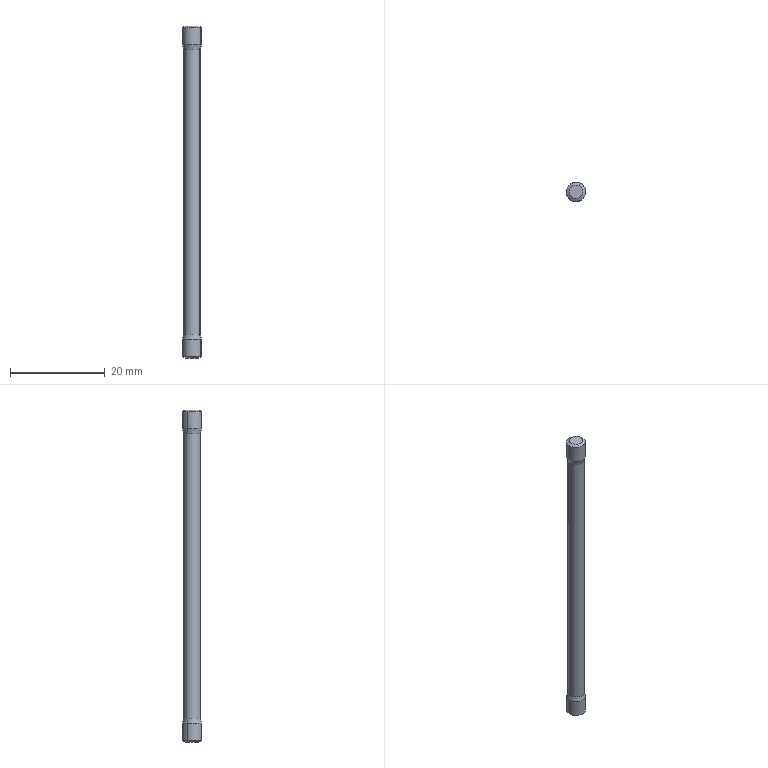Component | SolidWorks | GB_T901-1988EqualLengthDoubleEndStudGradeBM4x70-1 | 1 solid | 16 faces | box 4 x 4 x 70 mm | volume 685 mm3 | cone 8 | cylinder 6 | plane 2 | commonest cylinder face diameters 4 x4 3.464 x2
build123d program:
from build123d import *


with BuildPart() as part:
    # Sketch1 → Base-Revolve (revolve)
    with BuildSketch(Plane.XY, mode=Mode.PRIVATE) as base_revolve_sk:
        Polygon((-35, 2), (-31, 2), (-30.02, 1.732), (0, 1.732), (0, 0), (-35, 0), align=None)
    revolve(base_revolve_sk.sketch.rotate(Axis((-35, 0, 0), (1, 0, 0)), 180), axis=Axis((-35, 0, 0), (1, 0, 0)))

    # Sketch2 → Thread Cut (revolve, cut)
    with BuildSketch(Plane.XY, mode=Mode.PRIVATE) as thread_cut_sk:
        Polygon((-35.35, 2), (-34.65, 2), (-35, 1.394), align=None)
    revolve(thread_cut_sk.sketch.rotate(Axis((-26.952, 0, 0), (1, 0, 0)), 180), axis=Axis((-26.952, 0, 0), (1, 0, 0)), mode=Mode.SUBTRACT)

    # Mirror All1: part across plane


with BuildPart() as part_1:
    add(part.part)
    add(part.part.mirror(Plane(origin=(0, 1.732, 0), x_dir=(0, 0, 1), z_dir=(-1, 0, 0))))


solid = part_1.part

# Placed as in the assembly
solid = solid.moved(Location((-5.875, 10.354, 22.484), (0, 90, 0)))
STEP:
#1=COLOUR_RGB('',0.7922,0.8196,0.9333);
#2=FILL_AREA_STYLE_COLOUR('',#1);
#3=FILL_AREA_STYLE('',(#2));
#4=SURFACE_STYLE_FILL_AREA(#3);
#5=SURFACE_SIDE_STYLE('',(#4));
#6=SURFACE_STYLE_USAGE(.BOTH.,#5);
#7=PRESENTATION_STYLE_ASSIGNMENT((#6));
#8=CARTESIAN_POINT('',(-0.2571,0.3592,2.263));
#9=VERTEX_POINT('',#8);
#10=CARTESIAN_POINT('',(-0.2055,0.456,2.263));
#11=VERTEX_POINT('',#10);
#12=CARTESIAN_POINT('',(-0.2313,0.4076,2.263));
#13=DIRECTION('',(0.,0.,-1.));
#14=DIRECTION('',(0.4702,0.8826,0.));
#15=AXIS2_PLACEMENT_3D('',#12,#13,#14);
#16=CIRCLE('',#15,0.05487);
#17=EDGE_CURVE('',#9,#11,#16,.T.);
#18=ORIENTED_EDGE('',*,*,#17,.T.);
#19=CARTESIAN_POINT('',(-0.1943,0.4771,2.249));
#20=VERTEX_POINT('',#19);
#21=CARTESIAN_POINT('',(-0.2055,0.456,2.263));
#22=DIRECTION('',(0.4072,0.7643,-0.5));
#23=VECTOR('',#22,39.37);
#24=LINE('',#21,#23);
#25=EDGE_CURVE('',#11,#20,#24,.T.);
#26=ORIENTED_EDGE('',*,*,#25,.T.);
#27=CARTESIAN_POINT('',(-0.3008,0.4446,2.249));
#28=VERTEX_POINT('',#27);
#29=CARTESIAN_POINT('',(-0.2313,0.4076,2.249));
#30=DIRECTION('',(0.,0.,-1.));
#31=DIRECTION('',(0.4702,0.8826,0.));
#32=AXIS2_PLACEMENT_3D('',#29,#30,#31);
#33=CIRCLE('',#32,0.07874);
#34=EDGE_CURVE('',#28,#20,#33,.T.);
#35=ORIENTED_EDGE('',*,*,#34,.F.);
#36=CARTESIAN_POINT('',(-0.2683,0.3381,2.249));
#37=VERTEX_POINT('',#36);
#38=CARTESIAN_POINT('',(-0.2313,0.4076,2.249));
#39=DIRECTION('',(0.,0.,-1.));
#40=DIRECTION('',(0.4702,0.8826,0.));
#41=AXIS2_PLACEMENT_3D('',#38,#39,#40);
#42=CIRCLE('',#41,0.07874);
#43=EDGE_CURVE('',#37,#28,#42,.T.);
#44=ORIENTED_EDGE('',*,*,#43,.F.);
#45=CARTESIAN_POINT('',(-0.2571,0.3592,2.263));
#46=DIRECTION('',(-0.4072,-0.7643,-0.5));
#47=VECTOR('',#46,39.37);
#48=LINE('',#45,#47);
#49=EDGE_CURVE('',#9,#37,#48,.T.);
#50=ORIENTED_EDGE('',*,*,#49,.F.);
#51=EDGE_LOOP('',(#18,#26,#35,#44,#50));
#52=FACE_OUTER_BOUND('',#51,.T.);
#53=CARTESIAN_POINT('',(-0.2313,0.4076,2.263));
#54=DIRECTION('',(0.,0.,-1.));
#55=DIRECTION('',(-0.4702,-0.8826,0.));
#56=AXIS2_PLACEMENT_3D('',#53,#54,#55);
#57=CONICAL_SURFACE('',#56,0.05487,1.047);
#58=ADVANCED_FACE('',(#52),#57,.T.);
#59=CARTESIAN_POINT('',(-0.1711,0.3756,2.067));
#60=VERTEX_POINT('',#59);
#61=CARTESIAN_POINT('',(-0.2915,0.4397,2.067));
#62=VERTEX_POINT('',#61);
#63=CARTESIAN_POINT('',(-0.2313,0.4076,2.067));
#64=DIRECTION('',(0.,0.,-1.));
#65=DIRECTION('',(-0.8826,0.4702,0.));
#66=AXIS2_PLACEMENT_3D('',#63,#64,#65);
#67=CIRCLE('',#66,0.06819);
#68=EDGE_CURVE('',#60,#62,#67,.T.);
#69=ORIENTED_EDGE('',*,*,#68,.F.);
#70=CARTESIAN_POINT('',(-0.1618,0.3706,2.106));
#71=VERTEX_POINT('',#70);
#72=CARTESIAN_POINT('',(-0.1711,0.3756,2.067));
#73=DIRECTION('',(0.2328,-0.124,0.9646));
#74=VECTOR('',#73,39.37);
#75=LINE('',#72,#74);
#76=EDGE_CURVE('',#60,#71,#75,.T.);
#77=ORIENTED_EDGE('',*,*,#76,.T.);
#78=CARTESIAN_POINT('',(-0.3008,0.4446,2.106));
#79=VERTEX_POINT('',#78);
#80=CARTESIAN_POINT('',(-0.2313,0.4076,2.106));
#81=DIRECTION('',(0.,0.,-1.));
#82=DIRECTION('',(-0.8826,0.4702,0.));
#83=AXIS2_PLACEMENT_3D('',#80,#81,#82);
#84=CIRCLE('',#83,0.07874);
#85=EDGE_CURVE('',#71,#79,#84,.T.);
#86=ORIENTED_EDGE('',*,*,#85,.T.);
#87=CARTESIAN_POINT('',(-0.2915,0.4397,2.067));
#88=DIRECTION('',(-0.2328,0.124,0.9646));
#89=VECTOR('',#88,39.37);
#90=LINE('',#87,#89);
#91=EDGE_CURVE('',#62,#79,#90,.T.);
#92=ORIENTED_EDGE('',*,*,#91,.F.);
#93=EDGE_LOOP('',(#69,#77,#86,#92));
#94=FACE_OUTER_BOUND('',#93,.T.);
#95=CARTESIAN_POINT('',(-0.2313,0.4076,2.067));
#96=DIRECTION('',(-0.,-0.,1.));
#97=DIRECTION('',(-0.8826,0.4702,0.));
#98=AXIS2_PLACEMENT_3D('',#95,#96,#97);
#99=CONICAL_SURFACE('',#98,0.06819,0.2669);
#100=ADVANCED_FACE('',(#94),#99,.T.);
#101=ORIENTED_EDGE('',*,*,#85,.F.);
#102=CARTESIAN_POINT('',(-0.1618,0.3706,2.249));
#103=VERTEX_POINT('',#102);
#104=CARTESIAN_POINT('',(-0.1618,0.3706,2.263));
#105=DIRECTION('',(-0.,-0.,1.));
#106=VECTOR('',#105,39.37);
#107=LINE('',#104,#106);
#108=EDGE_CURVE('',#71,#103,#107,.T.);
#109=ORIENTED_EDGE('',*,*,#108,.T.);
#110=CARTESIAN_POINT('',(-0.2313,0.4076,2.249));
#111=DIRECTION('',(0.,0.,-1.));
#112=DIRECTION('',(0.4702,0.8826,0.));
#113=AXIS2_PLACEMENT_3D('',#110,#111,#112);
#114=CIRCLE('',#113,0.07874);
#115=EDGE_CURVE('',#103,#37,#114,.T.);
#116=ORIENTED_EDGE('',*,*,#115,.T.);
#117=ORIENTED_EDGE('',*,*,#43,.T.);
#118=CARTESIAN_POINT('',(-0.3008,0.4446,2.263));
#119=DIRECTION('',(-0.,-0.,1.));
#120=VECTOR('',#119,39.37);
#121=LINE('',#118,#120);
#122=EDGE_CURVE('',#79,#28,#121,.T.);
#123=ORIENTED_EDGE('',*,*,#122,.F.);
#124=EDGE_LOOP('',(#101,#109,#116,#117,#123));
#125=FACE_OUTER_BOUND('',#124,.T.);
#126=CARTESIAN_POINT('',(-0.2313,0.4076,2.263));
#127=DIRECTION('',(-0.,-0.,1.));
#128=DIRECTION('',(-0.8826,0.4702,0.));
#129=AXIS2_PLACEMENT_3D('',#126,#127,#128);
#130=CYLINDRICAL_SURFACE('',#129,0.07874);
#131=ADVANCED_FACE('',(#125),#130,.T.);
#132=CARTESIAN_POINT('',(-0.2055,0.456,-0.4928));
#133=VERTEX_POINT('',#132);
#134=CARTESIAN_POINT('',(-0.2571,0.3592,-0.4928));
#135=VERTEX_POINT('',#134);
#136=CARTESIAN_POINT('',(-0.2313,0.4076,-0.4928));
#137=DIRECTION('',(0.,0.,-1.));
#138=DIRECTION('',(0.4702,0.8826,0.));
#139=AXIS2_PLACEMENT_3D('',#136,#137,#138);
#140=CIRCLE('',#139,0.05487);
#141=EDGE_CURVE('',#133,#135,#140,.T.);
#142=ORIENTED_EDGE('',*,*,#141,.F.);
#143=CARTESIAN_POINT('',(-0.1943,0.4771,-0.479));
#144=VERTEX_POINT('',#143);
#145=CARTESIAN_POINT('',(-0.2055,0.456,-0.4928));
#146=DIRECTION('',(0.4072,0.7643,0.5));
#147=VECTOR('',#146,39.37);
#148=LINE('',#145,#147);
#149=EDGE_CURVE('',#133,#144,#148,.T.);
#150=ORIENTED_EDGE('',*,*,#149,.T.);
#151=CARTESIAN_POINT('',(-0.1618,0.3706,-0.479));
#152=VERTEX_POINT('',#151);
#153=CARTESIAN_POINT('',(-0.2313,0.4076,-0.479));
#154=DIRECTION('',(0.,0.,-1.));
#155=DIRECTION('',(0.4702,0.8826,0.));
#156=AXIS2_PLACEMENT_3D('',#153,#154,#155);
#157=CIRCLE('',#156,0.07874);
#158=EDGE_CURVE('',#144,#152,#157,.T.);
#159=ORIENTED_EDGE('',*,*,#158,.T.);
#160=CARTESIAN_POINT('',(-0.2683,0.3381,-0.479));
#161=VERTEX_POINT('',#160);
#162=CARTESIAN_POINT('',(-0.2313,0.4076,-0.479));
#163=DIRECTION('',(0.,0.,-1.));
#164=DIRECTION('',(0.4702,0.8826,0.));
#165=AXIS2_PLACEMENT_3D('',#162,#163,#164);
#166=CIRCLE('',#165,0.07874);
#167=EDGE_CURVE('',#152,#161,#166,.T.);
#168=ORIENTED_EDGE('',*,*,#167,.T.);
#169=CARTESIAN_POINT('',(-0.2571,0.3592,-0.4928));
#170=DIRECTION('',(-0.4072,-0.7643,0.5));
#171=VECTOR('',#170,39.37);
#172=LINE('',#169,#171);
#173=EDGE_CURVE('',#135,#161,#172,.T.);
#174=ORIENTED_EDGE('',*,*,#173,.F.);
#175=EDGE_LOOP('',(#142,#150,#159,#168,#174));
#176=FACE_OUTER_BOUND('',#175,.T.);
#177=CARTESIAN_POINT('',(-0.2313,0.4076,-0.4928));
#178=DIRECTION('',(-0.,-0.,1.));
#179=DIRECTION('',(-0.4702,-0.8826,0.));
#180=AXIS2_PLACEMENT_3D('',#177,#178,#179);
#181=CONICAL_SURFACE('',#180,0.05487,1.047);
#182=ADVANCED_FACE('',(#176),#181,.T.);
#183=CARTESIAN_POINT('',(-0.2915,0.4397,-0.2967));
#184=VERTEX_POINT('',#183);
#185=CARTESIAN_POINT('',(-0.1711,0.3756,-0.2967));
#186=VERTEX_POINT('',#185);
#187=CARTESIAN_POINT('',(-0.2313,0.4076,-0.2967));
#188=DIRECTION('',(0.,0.,-1.));
#189=DIRECTION('',(-0.8826,0.4702,0.));
#190=AXIS2_PLACEMENT_3D('',#187,#188,#189);
#191=CIRCLE('',#190,0.06819);
#192=EDGE_CURVE('',#184,#186,#191,.T.);
#193=ORIENTED_EDGE('',*,*,#192,.T.);
#194=CARTESIAN_POINT('',(-0.1618,0.3706,-0.3353));
#195=VERTEX_POINT('',#194);
#196=CARTESIAN_POINT('',(-0.1711,0.3756,-0.2967));
#197=DIRECTION('',(0.2328,-0.124,-0.9646));
#198=VECTOR('',#197,39.37);
#199=LINE('',#196,#198);
#200=EDGE_CURVE('',#186,#195,#199,.T.);
#201=ORIENTED_EDGE('',*,*,#200,.T.);
#202=CARTESIAN_POINT('',(-0.3008,0.4446,-0.3353));
#203=VERTEX_POINT('',#202);
#204=CARTESIAN_POINT('',(-0.2313,0.4076,-0.3353));
#205=DIRECTION('',(0.,0.,-1.));
#206=DIRECTION('',(-0.8826,0.4702,0.));
#207=AXIS2_PLACEMENT_3D('',#204,#205,#206);
#208=CIRCLE('',#207,0.07874);
#209=EDGE_CURVE('',#203,#195,#208,.T.);
#210=ORIENTED_EDGE('',*,*,#209,.F.);
#211=CARTESIAN_POINT('',(-0.2915,0.4397,-0.2967));
#212=DIRECTION('',(-0.2328,0.124,-0.9646));
#213=VECTOR('',#212,39.37);
#214=LINE('',#211,#213);
#215=EDGE_CURVE('',#184,#203,#214,.T.);
#216=ORIENTED_EDGE('',*,*,#215,.F.);
#217=EDGE_LOOP('',(#193,#201,#210,#216));
#218=FACE_OUTER_BOUND('',#217,.T.);
#219=CARTESIAN_POINT('',(-0.2313,0.4076,-0.2967));
#220=DIRECTION('',(0.,0.,-1.));
#221=DIRECTION('',(-0.8826,0.4702,0.));
#222=AXIS2_PLACEMENT_3D('',#219,#220,#221);
#223=CONICAL_SURFACE('',#222,0.06819,0.2669);
#224=ADVANCED_FACE('',(#218),#223,.T.);
#225=CARTESIAN_POINT('',(-0.2313,0.4076,2.067));
#226=DIRECTION('',(0.,0.,-1.));
#227=DIRECTION('',(-0.8826,0.4702,0.));
#228=AXIS2_PLACEMENT_3D('',#225,#226,#227);
#229=CIRCLE('',#228,0.06819);
#230=EDGE_CURVE('',#62,#60,#229,.T.);
#231=ORIENTED_EDGE('',*,*,#230,.T.);
#232=CARTESIAN_POINT('',(-0.1711,0.3756,-0.4928));
#233=DIRECTION('',(0.,0.,-1.));
#234=VECTOR('',#233,39.37);
#235=LINE('',#232,#234);
#236=EDGE_CURVE('',#60,#186,#235,.T.);
#237=ORIENTED_EDGE('',*,*,#236,.T.);
#238=ORIENTED_EDGE('',*,*,#192,.F.);
#239=CARTESIAN_POINT('',(-0.2915,0.4397,-0.4928));
#240=DIRECTION('',(0.,0.,-1.));
#241=VECTOR('',#240,39.37);
#242=LINE('',#239,#241);
#243=EDGE_CURVE('',#62,#184,#242,.T.);
#244=ORIENTED_EDGE('',*,*,#243,.F.);
#245=EDGE_LOOP('',(#231,#237,#238,#244));
#246=FACE_OUTER_BOUND('',#245,.T.);
#247=CARTESIAN_POINT('',(-0.2313,0.4076,-0.4928));
#248=DIRECTION('',(0.,0.,-1.));
#249=DIRECTION('',(-0.8826,0.4702,0.));
#250=AXIS2_PLACEMENT_3D('',#247,#248,#249);
#251=CYLINDRICAL_SURFACE('',#250,0.06819);
#252=ADVANCED_FACE('',(#246),#251,.T.);
#253=ORIENTED_EDGE('',*,*,#209,.T.);
#254=CARTESIAN_POINT('',(-0.1618,0.3706,-0.4928));
#255=DIRECTION('',(0.,0.,-1.));
#256=VECTOR('',#255,39.37);
#257=LINE('',#254,#256);
#258=EDGE_CURVE('',#195,#152,#257,.T.);
#259=ORIENTED_EDGE('',*,*,#258,.T.);
#260=ORIENTED_EDGE('',*,*,#158,.F.);
#261=CARTESIAN_POINT('',(-0.3008,0.4446,-0.479));
#262=VERTEX_POINT('',#261);
#263=CARTESIAN_POINT('',(-0.2313,0.4076,-0.479));
#264=DIRECTION('',(0.,0.,-1.));
#265=DIRECTION('',(0.4702,0.8826,0.));
#266=AXIS2_PLACEMENT_3D('',#263,#264,#265);
#267=CIRCLE('',#266,0.07874);
#268=EDGE_CURVE('',#262,#144,#267,.T.);
#269=ORIENTED_EDGE('',*,*,#268,.F.);
#270=CARTESIAN_POINT('',(-0.3008,0.4446,-0.4928));
#271=DIRECTION('',(0.,0.,-1.));
#272=VECTOR('',#271,39.37);
#273=LINE('',#270,#272);
#274=EDGE_CURVE('',#203,#262,#273,.T.);
#275=ORIENTED_EDGE('',*,*,#274,.F.);
#276=EDGE_LOOP('',(#253,#259,#260,#269,#275));
#277=FACE_OUTER_BOUND('',#276,.T.);
#278=CARTESIAN_POINT('',(-0.2313,0.4076,-0.4928));
#279=DIRECTION('',(0.,0.,-1.));
#280=DIRECTION('',(-0.8826,0.4702,0.));
#281=AXIS2_PLACEMENT_3D('',#278,#279,#280);
#282=CYLINDRICAL_SURFACE('',#281,0.07874);
#283=ADVANCED_FACE('',(#277),#282,.T.);
#284=ORIENTED_EDGE('',*,*,#258,.F.);
#285=CARTESIAN_POINT('',(-0.2313,0.4076,-0.3353));
#286=DIRECTION('',(0.,0.,-1.));
#287=DIRECTION('',(-0.8826,0.4702,0.));
#288=AXIS2_PLACEMENT_3D('',#285,#286,#287);
#289=CIRCLE('',#288,0.07874);
#290=EDGE_CURVE('',#195,#203,#289,.T.);
#291=ORIENTED_EDGE('',*,*,#290,.T.);
#292=ORIENTED_EDGE('',*,*,#274,.T.);
#293=CARTESIAN_POINT('',(-0.2313,0.4076,-0.479));
#294=DIRECTION('',(0.,0.,-1.));
#295=DIRECTION('',(0.4702,0.8826,0.));
#296=AXIS2_PLACEMENT_3D('',#293,#294,#295);
#297=CIRCLE('',#296,0.07874);
#298=EDGE_CURVE('',#161,#262,#297,.T.);
#299=ORIENTED_EDGE('',*,*,#298,.F.);
#300=ORIENTED_EDGE('',*,*,#167,.F.);
#301=EDGE_LOOP('',(#284,#291,#292,#299,#300));
#302=FACE_OUTER_BOUND('',#301,.T.);
#303=CARTESIAN_POINT('',(-0.2313,0.4076,-0.4928));
#304=DIRECTION('',(0.,0.,-1.));
#305=DIRECTION('',(-0.8826,0.4702,0.));
#306=AXIS2_PLACEMENT_3D('',#303,#304,#305);
#307=CYLINDRICAL_SURFACE('',#306,0.07874);
#308=ADVANCED_FACE('',(#302),#307,.T.);
#309=ORIENTED_EDGE('',*,*,#236,.F.);
#310=ORIENTED_EDGE('',*,*,#68,.T.);
#311=ORIENTED_EDGE('',*,*,#243,.T.);
#312=CARTESIAN_POINT('',(-0.2313,0.4076,-0.2967));
#313=DIRECTION('',(0.,0.,-1.));
#314=DIRECTION('',(-0.8826,0.4702,0.));
#315=AXIS2_PLACEMENT_3D('',#312,#313,#314);
#316=CIRCLE('',#315,0.06819);
#317=EDGE_CURVE('',#186,#184,#316,.T.);
#318=ORIENTED_EDGE('',*,*,#317,.F.);
#319=EDGE_LOOP('',(#309,#310,#311,#318));
#320=FACE_OUTER_BOUND('',#319,.T.);
#321=CARTESIAN_POINT('',(-0.2313,0.4076,-0.4928));
#322=DIRECTION('',(0.,0.,-1.));
#323=DIRECTION('',(-0.8826,0.4702,0.));
#324=AXIS2_PLACEMENT_3D('',#321,#322,#323);
#325=CYLINDRICAL_SURFACE('',#324,0.06819);
#326=ADVANCED_FACE('',(#320),#325,.T.);
#327=ORIENTED_EDGE('',*,*,#200,.F.);
#328=ORIENTED_EDGE('',*,*,#317,.T.);
#329=ORIENTED_EDGE('',*,*,#215,.T.);
#330=ORIENTED_EDGE('',*,*,#290,.F.);
#331=EDGE_LOOP('',(#327,#328,#329,#330));
#332=FACE_OUTER_BOUND('',#331,.T.);
#333=CARTESIAN_POINT('',(-0.2313,0.4076,-0.2967));
#334=DIRECTION('',(0.,0.,-1.));
#335=DIRECTION('',(-0.8826,0.4702,0.));
#336=AXIS2_PLACEMENT_3D('',#333,#334,#335);
#337=CONICAL_SURFACE('',#336,0.06819,0.2669);
#338=ADVANCED_FACE('',(#332),#337,.T.);
#339=ORIENTED_EDGE('',*,*,#149,.F.);
#340=CARTESIAN_POINT('',(-0.2313,0.4076,-0.4928));
#341=DIRECTION('',(0.,0.,-1.));
#342=DIRECTION('',(0.4702,0.8826,0.));
#343=AXIS2_PLACEMENT_3D('',#340,#341,#342);
#344=CIRCLE('',#343,0.05487);
#345=EDGE_CURVE('',#135,#133,#344,.T.);
#346=ORIENTED_EDGE('',*,*,#345,.F.);
#347=ORIENTED_EDGE('',*,*,#173,.T.);
#348=ORIENTED_EDGE('',*,*,#298,.T.);
#349=ORIENTED_EDGE('',*,*,#268,.T.);
#350=EDGE_LOOP('',(#339,#346,#347,#348,#349));
#351=FACE_OUTER_BOUND('',#350,.T.);
#352=CARTESIAN_POINT('',(-0.2313,0.4076,-0.4928));
#353=DIRECTION('',(-0.,-0.,1.));
#354=DIRECTION('',(-0.4702,-0.8826,0.));
#355=AXIS2_PLACEMENT_3D('',#352,#353,#354);
#356=CONICAL_SURFACE('',#355,0.05487,1.047);
#357=ADVANCED_FACE('',(#351),#356,.T.);
#358=ORIENTED_EDGE('',*,*,#345,.T.);
#359=ORIENTED_EDGE('',*,*,#141,.T.);
#360=EDGE_LOOP('',(#358,#359));
#361=FACE_OUTER_BOUND('',#360,.T.);
#362=CARTESIAN_POINT('',(-0.1618,0.3706,-0.4928));
#363=DIRECTION('',(-0.,-0.,1.));
#364=DIRECTION('',(0.8826,-0.4702,0.));
#365=AXIS2_PLACEMENT_3D('',#362,#363,#364);
#366=PLANE('',#365);
#367=ADVANCED_FACE('',(#361),#366,.F.);
#368=ORIENTED_EDGE('',*,*,#108,.F.);
#369=CARTESIAN_POINT('',(-0.2313,0.4076,2.106));
#370=DIRECTION('',(0.,0.,-1.));
#371=DIRECTION('',(-0.8826,0.4702,0.));
#372=AXIS2_PLACEMENT_3D('',#369,#370,#371);
#373=CIRCLE('',#372,0.07874);
#374=EDGE_CURVE('',#79,#71,#373,.T.);
#375=ORIENTED_EDGE('',*,*,#374,.F.);
#376=ORIENTED_EDGE('',*,*,#122,.T.);
#377=ORIENTED_EDGE('',*,*,#34,.T.);
#378=CARTESIAN_POINT('',(-0.2313,0.4076,2.249));
#379=DIRECTION('',(0.,0.,-1.));
#380=DIRECTION('',(0.4702,0.8826,0.));
#381=AXIS2_PLACEMENT_3D('',#378,#379,#380);
#382=CIRCLE('',#381,0.07874);
#383=EDGE_CURVE('',#20,#103,#382,.T.);
#384=ORIENTED_EDGE('',*,*,#383,.T.);
#385=EDGE_LOOP('',(#368,#375,#376,#377,#384));
#386=FACE_OUTER_BOUND('',#385,.T.);
#387=CARTESIAN_POINT('',(-0.2313,0.4076,2.263));
#388=DIRECTION('',(-0.,-0.,1.));
#389=DIRECTION('',(-0.8826,0.4702,0.));
#390=AXIS2_PLACEMENT_3D('',#387,#388,#389);
#391=CYLINDRICAL_SURFACE('',#390,0.07874);
#392=ADVANCED_FACE('',(#386),#391,.T.);
#393=ORIENTED_EDGE('',*,*,#76,.F.);
#394=ORIENTED_EDGE('',*,*,#230,.F.);
#395=ORIENTED_EDGE('',*,*,#91,.T.);
#396=ORIENTED_EDGE('',*,*,#374,.T.);
#397=EDGE_LOOP('',(#393,#394,#395,#396));
#398=FACE_OUTER_BOUND('',#397,.T.);
#399=CARTESIAN_POINT('',(-0.2313,0.4076,2.067));
#400=DIRECTION('',(-0.,-0.,1.));
#401=DIRECTION('',(-0.8826,0.4702,0.));
#402=AXIS2_PLACEMENT_3D('',#399,#400,#401);
#403=CONICAL_SURFACE('',#402,0.06819,0.2669);
#404=ADVANCED_FACE('',(#398),#403,.T.);
#405=ORIENTED_EDGE('',*,*,#25,.F.);
#406=CARTESIAN_POINT('',(-0.2313,0.4076,2.263));
#407=DIRECTION('',(0.,0.,-1.));
#408=DIRECTION('',(0.4702,0.8826,0.));
#409=AXIS2_PLACEMENT_3D('',#406,#407,#408);
#410=CIRCLE('',#409,0.05487);
#411=EDGE_CURVE('',#11,#9,#410,.T.);
#412=ORIENTED_EDGE('',*,*,#411,.T.);
#413=ORIENTED_EDGE('',*,*,#49,.T.);
#414=ORIENTED_EDGE('',*,*,#115,.F.);
#415=ORIENTED_EDGE('',*,*,#383,.F.);
#416=EDGE_LOOP('',(#405,#412,#413,#414,#415));
#417=FACE_OUTER_BOUND('',#416,.T.);
#418=CARTESIAN_POINT('',(-0.2313,0.4076,2.263));
#419=DIRECTION('',(0.,0.,-1.));
#420=DIRECTION('',(-0.4702,-0.8826,0.));
#421=AXIS2_PLACEMENT_3D('',#418,#419,#420);
#422=CONICAL_SURFACE('',#421,0.05487,1.047);
#423=ADVANCED_FACE('',(#417),#422,.T.);
#424=ORIENTED_EDGE('',*,*,#17,.F.);
#425=ORIENTED_EDGE('',*,*,#411,.F.);
#426=EDGE_LOOP('',(#424,#425));
#427=FACE_OUTER_BOUND('',#426,.T.);
#428=CARTESIAN_POINT('',(-0.1618,0.3706,2.263));
#429=DIRECTION('',(0.,0.,-1.));
#430=DIRECTION('',(0.8826,-0.4702,0.));
#431=AXIS2_PLACEMENT_3D('',#428,#429,#430);
#432=PLANE('',#431);
#433=ADVANCED_FACE('',(#427),#432,.F.);
#434=CLOSED_SHELL('',(#58,#100,#131,#182,#224,#252,#283,#308,#326,#338,#357,#367,#392,#404,#423,#433));
#435=MANIFOLD_SOLID_BREP('',#434);
#436=STYLED_ITEM('',(#7),#435);
#437=(LENGTH_UNIT()NAMED_UNIT(*)SI_UNIT($,.METRE.));
#438=LENGTH_MEASURE_WITH_UNIT(LENGTH_MEASURE(0.0254),#437);
#439=DIMENSIONAL_EXPONENTS(1.,0.,0.,0.,0.,0.,0.);
#440=(CONVERSION_BASED_UNIT('',#438)LENGTH_UNIT()NAMED_UNIT(#439));
#441=UNCERTAINTY_MEASURE_WITH_UNIT(LENGTH_MEASURE(0.00001),#440,'','');
#442=(NAMED_UNIT(*)PLANE_ANGLE_UNIT()SI_UNIT($,.RADIAN.));
#443=(NAMED_UNIT(*)SI_UNIT($,.STERADIAN.)SOLID_ANGLE_UNIT());
#444=(GEOMETRIC_REPRESENTATION_CONTEXT(3)GLOBAL_UNCERTAINTY_ASSIGNED_CONTEXT((#441))GLOBAL_UNIT_ASSIGNED_CONTEXT((#440,#442,#443))REPRESENTATION_CONTEXT('',''));
#445=MECHANICAL_DESIGN_GEOMETRIC_PRESENTATION_REPRESENTATION('',(#436),#444);
#446=CARTESIAN_POINT('',(0.,0.,0.));
#447=DIRECTION('',(0.,0.,1.));
#448=DIRECTION('',(1.,0.,0.));
#449=AXIS2_PLACEMENT_3D('',#446,#447,#448);
#450=(LENGTH_UNIT()NAMED_UNIT(*)SI_UNIT($,.METRE.));
#451=LENGTH_MEASURE_WITH_UNIT(LENGTH_MEASURE(0.0254),#450);
#452=DIMENSIONAL_EXPONENTS(1.,0.,0.,0.,0.,0.,0.);
#453=(CONVERSION_BASED_UNIT('',#451)LENGTH_UNIT()NAMED_UNIT(#452));
#454=UNCERTAINTY_MEASURE_WITH_UNIT(LENGTH_MEASURE(0.00001),#453,'','');
#455=(NAMED_UNIT(*)PLANE_ANGLE_UNIT()SI_UNIT($,.RADIAN.));
#456=(NAMED_UNIT(*)SI_UNIT($,.STERADIAN.)SOLID_ANGLE_UNIT());
#457=(GEOMETRIC_REPRESENTATION_CONTEXT(3)GLOBAL_UNCERTAINTY_ASSIGNED_CONTEXT((#454))GLOBAL_UNIT_ASSIGNED_CONTEXT((#453,#455,#456))REPRESENTATION_CONTEXT('',''));
#458=ADVANCED_BREP_SHAPE_REPRESENTATION('',(#435,#449),#457);
#459=PRESENTATION_LAYER_ASSIGNMENT('','',(#436));